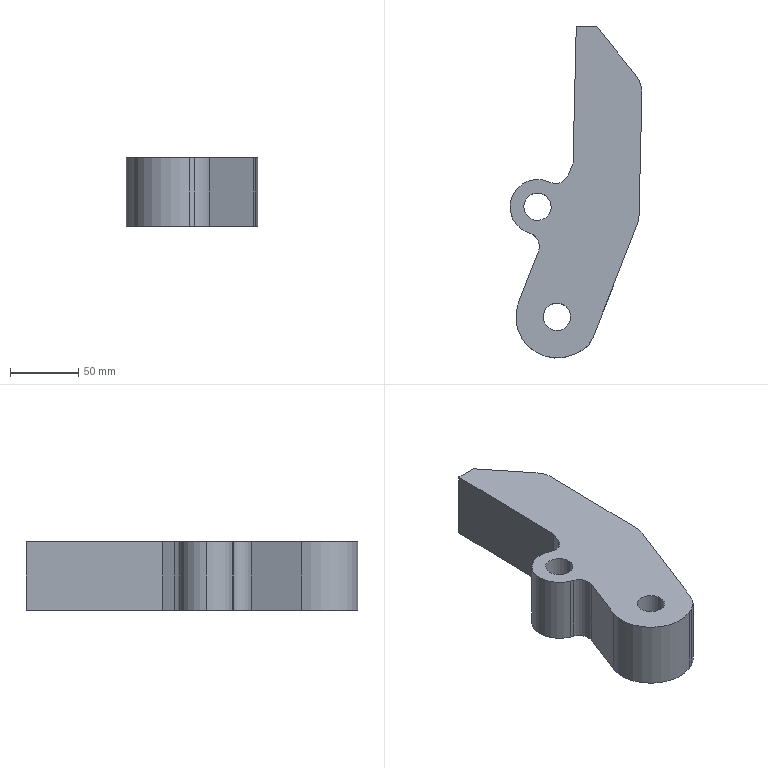Component | SolidWorks | BoxDoorCard-1 | 1 solid | 24 faces | box 96.24 x 242.36 x 50 mm | volume 653401 mm3 | cylinder 12 | plane 12 | commonest cylinder face diameters 20 x6 40 x5 60 x1
build123d program:
from build123d import *

# Parameters (mm, degrees)
BOSS_EXTRUDE1_DEPTH = 50
BOSS_EXTRUDE2_DEPTH = 50
FILLET1_R           = 10
FILLET2_R           = 20
SKETCH3_R           = 10
CUT_EXTRUDE1_DEPTH  = 255.94
SKETCH4_R           = 10
CUT_EXTRUDE2_DEPTH  = 50


with BuildPart() as part:
    # Sketch1 → Boss-Extrude1 (new body)
    with BuildSketch(Plane.XY):
        with BuildLine():
            Line((0, 0), (15, 0))
            Line((15, 0), (15, -100))
            Line((15, -100), (52.262, -202.376))
            ThreePointArc((52.262, -202.376), (44.339, -234.755), (11.393, -239.826))
            Line((11.393, -239.826), (0.1304, -234.574))
            Line((0.1304, -234.574), (-34.072, -140.605))
            Line((-34.072, -140.605), (-34.072, -40.605))
            Line((-34.072, -40.605), (0, 0))
        make_face()
    extrude(amount=BOSS_EXTRUDE1_DEPTH)

    # Sketch2 → Boss-Extrude2 (add)
    with BuildSketch(Plane.XY.offset(50)):
        with BuildLine():
            Line((21.594, -118.118), (33.341, -113.843))
            ThreePointArc((33.341, -113.843), (58.975, -125.796), (47.021, -151.431))
            Line((47.021, -151.431), (35.275, -155.706))
            Line((35.275, -155.706), (21.594, -118.118))
        make_face()
    extrude(amount=-BOSS_EXTRUDE2_DEPTH)

    # Fillet1
    fillet1_edges = [part.edges().sort_by_distance(p)[0] for p in [
        (35.275, -155.706, 25),
        (21.594, -118.118, 25),
    ]]
    fillet(fillet1_edges, radius=FILLET1_R)

    # Fillet2
    fillet2_edges = [part.edges().sort_by_distance(p)[0] for p in [
        (0.1304, -234.574, 25),
        (-34.072, -140.605, 25),
        (-34.072, -40.605, 25),
    ]]
    fillet(fillet2_edges, radius=FILLET2_R)

    # Sketch3 → Cut-Extrude1 (cut, through all)
    with BuildSketch(Plane.XY.offset(50)):
        with Locations((40.181, -132.637)):
            Circle(SKETCH3_R)
    extrude(amount=-CUT_EXTRUDE1_DEPTH, mode=Mode.SUBTRACT)

    # Sketch4 → Cut-Extrude2 (cut)
    with BuildSketch(Plane.XY.offset(50)):
        with Locations((24.071, -212.637)):
            Circle(SKETCH4_R)
    extrude(amount=-CUT_EXTRUDE2_DEPTH, mode=Mode.SUBTRACT)


solid = part.part

# Placed as in the assembly
solid = solid.moved(Location((1159.9, 1474.284, 520.114), (180, 0, -178.644)))
STEP:
#1=COLOUR_RGB('',0.7922,0.8196,0.9333);
#2=FILL_AREA_STYLE_COLOUR('',#1);
#3=FILL_AREA_STYLE('',(#2));
#4=SURFACE_STYLE_FILL_AREA(#3);
#5=SURFACE_SIDE_STYLE('',(#4));
#6=SURFACE_STYLE_USAGE(.BOTH.,#5);
#7=PRESENTATION_STYLE_ASSIGNMENT((#6));
#8=CARTESIAN_POINT('',(44.913,49.687,20.477));
#9=VERTEX_POINT('',#8);
#10=CARTESIAN_POINT('',(44.126,49.705,20.477));
#11=VERTEX_POINT('',#10);
#12=CARTESIAN_POINT('',(44.52,49.696,20.477));
#13=DIRECTION('',(-0.,-0.,-1.));
#14=DIRECTION('',(-0.9997,0.02366,0.));
#15=AXIS2_PLACEMENT_3D('',#12,#13,#14);
#16=CIRCLE('',#15,0.3937);
#17=EDGE_CURVE('',#9,#11,#16,.T.);
#18=ORIENTED_EDGE('',*,*,#17,.F.);
#19=CARTESIAN_POINT('',(44.913,49.687,18.508));
#20=VERTEX_POINT('',#19);
#21=CARTESIAN_POINT('',(44.913,49.687,20.477));
#22=DIRECTION('',(-0.,-0.,-1.));
#23=VECTOR('',#22,39.37);
#24=LINE('',#21,#23);
#25=EDGE_CURVE('',#9,#20,#24,.T.);
#26=ORIENTED_EDGE('',*,*,#25,.T.);
#27=CARTESIAN_POINT('',(44.126,49.705,18.508));
#28=VERTEX_POINT('',#27);
#29=CARTESIAN_POINT('',(44.52,49.696,18.508));
#30=DIRECTION('',(-0.,-0.,-1.));
#31=DIRECTION('',(-0.9997,0.02366,0.));
#32=AXIS2_PLACEMENT_3D('',#29,#30,#31);
#33=CIRCLE('',#32,0.3937);
#34=EDGE_CURVE('',#20,#28,#33,.T.);
#35=ORIENTED_EDGE('',*,*,#34,.T.);
#36=CARTESIAN_POINT('',(44.126,49.705,20.477));
#37=DIRECTION('',(-0.,-0.,-1.));
#38=VECTOR('',#37,39.37);
#39=LINE('',#36,#38);
#40=EDGE_CURVE('',#11,#28,#39,.T.);
#41=ORIENTED_EDGE('',*,*,#40,.F.);
#42=EDGE_LOOP('',(#18,#26,#35,#41));
#43=FACE_OUTER_BOUND('',#42,.T.);
#44=CARTESIAN_POINT('',(44.52,49.696,20.477));
#45=DIRECTION('',(-0.,-0.,-1.));
#46=DIRECTION('',(-0.9997,0.02366,0.));
#47=AXIS2_PLACEMENT_3D('',#44,#45,#46);
#48=CYLINDRICAL_SURFACE('',#47,0.3937);
#49=ADVANCED_FACE('',(#43),#48,.F.);
#50=CARTESIAN_POINT('',(44.354,52.85,20.477));
#51=VERTEX_POINT('',#50);
#52=CARTESIAN_POINT('',(43.567,52.869,20.477));
#53=VERTEX_POINT('',#52);
#54=CARTESIAN_POINT('',(43.96,52.86,20.477));
#55=DIRECTION('',(-0.,-0.,-1.));
#56=DIRECTION('',(-0.9997,0.02366,0.));
#57=AXIS2_PLACEMENT_3D('',#54,#55,#56);
#58=CIRCLE('',#57,0.3937);
#59=EDGE_CURVE('',#51,#53,#58,.T.);
#60=ORIENTED_EDGE('',*,*,#59,.F.);
#61=CARTESIAN_POINT('',(44.354,52.85,18.508));
#62=VERTEX_POINT('',#61);
#63=CARTESIAN_POINT('',(44.354,52.85,20.477));
#64=DIRECTION('',(-0.,-0.,-1.));
#65=VECTOR('',#64,39.37);
#66=LINE('',#63,#65);
#67=EDGE_CURVE('',#51,#62,#66,.T.);
#68=ORIENTED_EDGE('',*,*,#67,.T.);
#69=CARTESIAN_POINT('',(43.567,52.869,18.508));
#70=VERTEX_POINT('',#69);
#71=CARTESIAN_POINT('',(43.96,52.86,18.508));
#72=DIRECTION('',(-0.,-0.,-1.));
#73=DIRECTION('',(-0.9997,0.02366,0.));
#74=AXIS2_PLACEMENT_3D('',#71,#72,#73);
#75=CIRCLE('',#74,0.3937);
#76=EDGE_CURVE('',#62,#70,#75,.T.);
#77=ORIENTED_EDGE('',*,*,#76,.T.);
#78=CARTESIAN_POINT('',(43.567,52.869,20.477));
#79=DIRECTION('',(-0.,-0.,-1.));
#80=VECTOR('',#79,39.37);
#81=LINE('',#78,#80);
#82=EDGE_CURVE('',#53,#70,#81,.T.);
#83=ORIENTED_EDGE('',*,*,#82,.F.);
#84=EDGE_LOOP('',(#60,#68,#77,#83));
#85=FACE_OUTER_BOUND('',#84,.T.);
#86=CARTESIAN_POINT('',(43.96,52.86,20.477));
#87=DIRECTION('',(-0.,-0.,-1.));
#88=DIRECTION('',(-0.9997,0.02366,0.));
#89=AXIS2_PLACEMENT_3D('',#86,#87,#88);
#90=CYLINDRICAL_SURFACE('',#89,0.3937);
#91=ADVANCED_FACE('',(#85),#90,.F.);
#92=CARTESIAN_POINT('',(43.674,52.126,20.477));
#93=VERTEX_POINT('',#92);
#94=CARTESIAN_POINT('',(43.173,52.878,20.477));
#95=VERTEX_POINT('',#94);
#96=CARTESIAN_POINT('',(43.96,52.86,20.477));
#97=DIRECTION('',(-0.,-0.,-1.));
#98=DIRECTION('',(-0.9997,0.02366,0.));
#99=AXIS2_PLACEMENT_3D('',#96,#97,#98);
#100=CIRCLE('',#99,0.7874);
#101=EDGE_CURVE('',#93,#95,#100,.T.);
#102=ORIENTED_EDGE('',*,*,#101,.T.);
#103=CARTESIAN_POINT('',(43.173,52.878,18.508));
#104=VERTEX_POINT('',#103);
#105=CARTESIAN_POINT('',(43.173,52.878,20.477));
#106=DIRECTION('',(-0.,-0.,-1.));
#107=VECTOR('',#106,39.37);
#108=LINE('',#105,#107);
#109=EDGE_CURVE('',#95,#104,#108,.T.);
#110=ORIENTED_EDGE('',*,*,#109,.T.);
#111=CARTESIAN_POINT('',(43.674,52.126,18.508));
#112=VERTEX_POINT('',#111);
#113=CARTESIAN_POINT('',(43.96,52.86,18.508));
#114=DIRECTION('',(-0.,-0.,-1.));
#115=DIRECTION('',(-0.9997,0.02366,0.));
#116=AXIS2_PLACEMENT_3D('',#113,#114,#115);
#117=CIRCLE('',#116,0.7874);
#118=EDGE_CURVE('',#112,#104,#117,.T.);
#119=ORIENTED_EDGE('',*,*,#118,.F.);
#120=CARTESIAN_POINT('',(43.674,52.126,20.477));
#121=DIRECTION('',(-0.,-0.,-1.));
#122=VECTOR('',#121,39.37);
#123=LINE('',#120,#122);
#124=EDGE_CURVE('',#93,#112,#123,.T.);
#125=ORIENTED_EDGE('',*,*,#124,.F.);
#126=EDGE_LOOP('',(#102,#110,#119,#125));
#127=FACE_OUTER_BOUND('',#126,.T.);
#128=CARTESIAN_POINT('',(43.96,52.86,20.477));
#129=DIRECTION('',(-0.,-0.,-1.));
#130=DIRECTION('',(-0.9997,0.02366,0.));
#131=AXIS2_PLACEMENT_3D('',#128,#129,#130);
#132=CYLINDRICAL_SURFACE('',#131,0.7874);
#133=ADVANCED_FACE('',(#127),#132,.T.);
#134=CARTESIAN_POINT('',(44.849,53.78,18.508));
#135=VERTEX_POINT('',#134);
#136=CARTESIAN_POINT('',(44.982,54.121,18.508));
#137=VERTEX_POINT('',#136);
#138=CARTESIAN_POINT('',(44.982,54.121,18.508));
#139=DIRECTION('',(0.3642,0.9313,-0.));
#140=VECTOR('',#139,39.37);
#141=LINE('',#138,#140);
#142=EDGE_CURVE('',#135,#137,#141,.T.);
#143=ORIENTED_EDGE('',*,*,#142,.F.);
#144=CARTESIAN_POINT('',(44.849,53.78,20.477));
#145=VERTEX_POINT('',#144);
#146=CARTESIAN_POINT('',(44.849,53.78,18.508));
#147=DIRECTION('',(0.,0.,1.));
#148=VECTOR('',#147,39.37);
#149=LINE('',#146,#148);
#150=EDGE_CURVE('',#135,#145,#149,.T.);
#151=ORIENTED_EDGE('',*,*,#150,.T.);
#152=CARTESIAN_POINT('',(44.982,54.121,20.477));
#153=VERTEX_POINT('',#152);
#154=CARTESIAN_POINT('',(44.982,54.121,20.477));
#155=DIRECTION('',(0.3642,0.9313,-0.));
#156=VECTOR('',#155,39.37);
#157=LINE('',#154,#156);
#158=EDGE_CURVE('',#145,#153,#157,.T.);
#159=ORIENTED_EDGE('',*,*,#158,.T.);
#160=CARTESIAN_POINT('',(44.982,54.121,18.508));
#161=DIRECTION('',(0.,0.,1.));
#162=VECTOR('',#161,39.37);
#163=LINE('',#160,#162);
#164=EDGE_CURVE('',#137,#153,#163,.T.);
#165=ORIENTED_EDGE('',*,*,#164,.F.);
#166=EDGE_LOOP('',(#143,#151,#159,#165));
#167=FACE_OUTER_BOUND('',#166,.T.);
#168=CARTESIAN_POINT('',(44.982,54.121,18.508));
#169=DIRECTION('',(0.9313,-0.3642,-0.));
#170=DIRECTION('',(-0.3642,-0.9313,0.));
#171=AXIS2_PLACEMENT_3D('',#168,#169,#170);
#172=PLANE('',#171);
#173=ADVANCED_FACE('',(#167),#172,.F.);
#174=CARTESIAN_POINT('',(45.665,58.043,20.477));
#175=VERTEX_POINT('',#174);
#176=CARTESIAN_POINT('',(46.79,56.637,20.477));
#177=VERTEX_POINT('',#176);
#178=CARTESIAN_POINT('',(46.969,56.413,20.477));
#179=DIRECTION('',(0.6245,-0.781,0.));
#180=VECTOR('',#179,39.37);
#181=LINE('',#178,#180);
#182=EDGE_CURVE('',#175,#177,#181,.T.);
#183=ORIENTED_EDGE('',*,*,#182,.T.);
#184=CARTESIAN_POINT('',(46.79,56.637,18.508));
#185=VERTEX_POINT('',#184);
#186=CARTESIAN_POINT('',(46.79,56.637,18.508));
#187=DIRECTION('',(-0.,-0.,-1.));
#188=VECTOR('',#187,39.37);
#189=LINE('',#186,#188);
#190=EDGE_CURVE('',#177,#185,#189,.T.);
#191=ORIENTED_EDGE('',*,*,#190,.T.);
#192=CARTESIAN_POINT('',(45.665,58.043,18.508));
#193=VERTEX_POINT('',#192);
#194=CARTESIAN_POINT('',(46.969,56.413,18.508));
#195=DIRECTION('',(0.6245,-0.781,0.));
#196=VECTOR('',#195,39.37);
#197=LINE('',#194,#196);
#198=EDGE_CURVE('',#193,#185,#197,.T.);
#199=ORIENTED_EDGE('',*,*,#198,.F.);
#200=CARTESIAN_POINT('',(45.665,58.043,18.508));
#201=DIRECTION('',(0.,0.,1.));
#202=VECTOR('',#201,39.37);
#203=LINE('',#200,#202);
#204=EDGE_CURVE('',#193,#175,#203,.T.);
#205=ORIENTED_EDGE('',*,*,#204,.T.);
#206=EDGE_LOOP('',(#183,#191,#199,#205));
#207=FACE_OUTER_BOUND('',#206,.T.);
#208=CARTESIAN_POINT('',(46.969,56.413,18.508));
#209=DIRECTION('',(-0.781,-0.6245,0.));
#210=DIRECTION('',(-0.6245,0.781,-0.));
#211=AXIS2_PLACEMENT_3D('',#208,#209,#210);
#212=PLANE('',#211);
#213=ADVANCED_FACE('',(#207),#212,.F.);
#214=CARTESIAN_POINT('',(46.962,56.126,20.477));
#215=VERTEX_POINT('',#214);
#216=CARTESIAN_POINT('',(46.879,52.616,20.477));
#217=VERTEX_POINT('',#216);
#218=CARTESIAN_POINT('',(46.875,52.477,20.477));
#219=DIRECTION('',(-0.02366,-0.9997,0.));
#220=VECTOR('',#219,39.37);
#221=LINE('',#218,#220);
#222=EDGE_CURVE('',#215,#217,#221,.T.);
#223=ORIENTED_EDGE('',*,*,#222,.T.);
#224=CARTESIAN_POINT('',(46.879,52.616,18.508));
#225=VERTEX_POINT('',#224);
#226=CARTESIAN_POINT('',(46.879,52.616,18.508));
#227=DIRECTION('',(-0.,-0.,-1.));
#228=VECTOR('',#227,39.37);
#229=LINE('',#226,#228);
#230=EDGE_CURVE('',#217,#225,#229,.T.);
#231=ORIENTED_EDGE('',*,*,#230,.T.);
#232=CARTESIAN_POINT('',(46.962,56.126,18.508));
#233=VERTEX_POINT('',#232);
#234=CARTESIAN_POINT('',(46.875,52.477,18.508));
#235=DIRECTION('',(-0.02366,-0.9997,0.));
#236=VECTOR('',#235,39.37);
#237=LINE('',#234,#236);
#238=EDGE_CURVE('',#233,#225,#237,.T.);
#239=ORIENTED_EDGE('',*,*,#238,.F.);
#240=CARTESIAN_POINT('',(46.962,56.126,18.508));
#241=DIRECTION('',(0.,0.,1.));
#242=VECTOR('',#241,39.37);
#243=LINE('',#240,#242);
#244=EDGE_CURVE('',#233,#215,#243,.T.);
#245=ORIENTED_EDGE('',*,*,#244,.T.);
#246=EDGE_LOOP('',(#223,#231,#239,#245));
#247=FACE_OUTER_BOUND('',#246,.T.);
#248=CARTESIAN_POINT('',(46.875,52.477,18.508));
#249=DIRECTION('',(-0.9997,0.02366,0.));
#250=DIRECTION('',(0.,0.,1.));
#251=AXIS2_PLACEMENT_3D('',#248,#249,#250);
#252=PLANE('',#251);
#253=ADVANCED_FACE('',(#247),#252,.F.);
#254=CARTESIAN_POINT('',(46.825,52.348,20.477));
#255=VERTEX_POINT('',#254);
#256=CARTESIAN_POINT('',(45.56,49.114,20.477));
#257=VERTEX_POINT('',#256);
#258=CARTESIAN_POINT('',(45.442,48.81,20.477));
#259=DIRECTION('',(-0.3642,-0.9313,0.));
#260=VECTOR('',#259,39.37);
#261=LINE('',#258,#260);
#262=EDGE_CURVE('',#255,#257,#261,.T.);
#263=ORIENTED_EDGE('',*,*,#262,.T.);
#264=CARTESIAN_POINT('',(45.56,49.114,18.508));
#265=VERTEX_POINT('',#264);
#266=CARTESIAN_POINT('',(45.56,49.114,18.508));
#267=DIRECTION('',(-0.,-0.,-1.));
#268=VECTOR('',#267,39.37);
#269=LINE('',#266,#268);
#270=EDGE_CURVE('',#257,#265,#269,.T.);
#271=ORIENTED_EDGE('',*,*,#270,.T.);
#272=CARTESIAN_POINT('',(46.825,52.348,18.508));
#273=VERTEX_POINT('',#272);
#274=CARTESIAN_POINT('',(45.442,48.81,18.508));
#275=DIRECTION('',(-0.3642,-0.9313,0.));
#276=VECTOR('',#275,39.37);
#277=LINE('',#274,#276);
#278=EDGE_CURVE('',#273,#265,#277,.T.);
#279=ORIENTED_EDGE('',*,*,#278,.F.);
#280=CARTESIAN_POINT('',(46.825,52.348,18.508));
#281=DIRECTION('',(0.,0.,1.));
#282=VECTOR('',#281,39.37);
#283=LINE('',#280,#282);
#284=EDGE_CURVE('',#273,#255,#283,.T.);
#285=ORIENTED_EDGE('',*,*,#284,.T.);
#286=EDGE_LOOP('',(#263,#271,#279,#285));
#287=FACE_OUTER_BOUND('',#286,.T.);
#288=CARTESIAN_POINT('',(45.442,48.81,18.508));
#289=DIRECTION('',(-0.9313,0.3642,0.));
#290=DIRECTION('',(0.3642,0.9313,-0.));
#291=AXIS2_PLACEMENT_3D('',#288,#289,#290);
#292=PLANE('',#291);
#293=ADVANCED_FACE('',(#287),#292,.F.);
#294=CARTESIAN_POINT('',(45.143,48.679,18.508));
#295=VERTEX_POINT('',#294);
#296=CARTESIAN_POINT('',(44.994,48.614,18.508));
#297=VERTEX_POINT('',#296);
#298=CARTESIAN_POINT('',(44.994,48.614,18.508));
#299=DIRECTION('',(-0.9161,-0.4011,0.));
#300=VECTOR('',#299,39.37);
#301=LINE('',#298,#300);
#302=EDGE_CURVE('',#295,#297,#301,.T.);
#303=ORIENTED_EDGE('',*,*,#302,.F.);
#304=CARTESIAN_POINT('',(45.143,48.679,20.477));
#305=VERTEX_POINT('',#304);
#306=CARTESIAN_POINT('',(45.143,48.679,18.508));
#307=DIRECTION('',(0.,0.,1.));
#308=VECTOR('',#307,39.37);
#309=LINE('',#306,#308);
#310=EDGE_CURVE('',#295,#305,#309,.T.);
#311=ORIENTED_EDGE('',*,*,#310,.T.);
#312=CARTESIAN_POINT('',(44.994,48.614,20.477));
#313=VERTEX_POINT('',#312);
#314=CARTESIAN_POINT('',(44.994,48.614,20.477));
#315=DIRECTION('',(-0.9161,-0.4011,0.));
#316=VECTOR('',#315,39.37);
#317=LINE('',#314,#316);
#318=EDGE_CURVE('',#305,#313,#317,.T.);
#319=ORIENTED_EDGE('',*,*,#318,.T.);
#320=CARTESIAN_POINT('',(44.994,48.614,18.508));
#321=DIRECTION('',(0.,0.,1.));
#322=VECTOR('',#321,39.37);
#323=LINE('',#320,#322);
#324=EDGE_CURVE('',#297,#313,#323,.T.);
#325=ORIENTED_EDGE('',*,*,#324,.F.);
#326=EDGE_LOOP('',(#303,#311,#319,#325));
#327=FACE_OUTER_BOUND('',#326,.T.);
#328=CARTESIAN_POINT('',(44.994,48.614,18.508));
#329=DIRECTION('',(-0.4011,0.9161,-0.));
#330=DIRECTION('',(0.9161,0.4011,-0.));
#331=AXIS2_PLACEMENT_3D('',#328,#329,#330);
#332=PLANE('',#331);
#333=ADVANCED_FACE('',(#327),#332,.F.);
#334=CARTESIAN_POINT('',(43.42,50.126,20.477));
#335=VERTEX_POINT('',#334);
#336=CARTESIAN_POINT('',(44.52,49.696,20.477));
#337=DIRECTION('',(-0.,-0.,-1.));
#338=DIRECTION('',(0.9997,-0.02366,0.));
#339=AXIS2_PLACEMENT_3D('',#336,#337,#338);
#340=CIRCLE('',#339,1.181);
#341=EDGE_CURVE('',#313,#335,#340,.T.);
#342=ORIENTED_EDGE('',*,*,#341,.T.);
#343=CARTESIAN_POINT('',(43.42,50.126,18.508));
#344=VERTEX_POINT('',#343);
#345=CARTESIAN_POINT('',(43.42,50.126,18.508));
#346=DIRECTION('',(0.,0.,1.));
#347=VECTOR('',#346,39.37);
#348=LINE('',#345,#347);
#349=EDGE_CURVE('',#344,#335,#348,.T.);
#350=ORIENTED_EDGE('',*,*,#349,.F.);
#351=CARTESIAN_POINT('',(44.52,49.696,18.508));
#352=DIRECTION('',(-0.,-0.,-1.));
#353=DIRECTION('',(0.9997,-0.02366,0.));
#354=AXIS2_PLACEMENT_3D('',#351,#352,#353);
#355=CIRCLE('',#354,1.181);
#356=EDGE_CURVE('',#297,#344,#355,.T.);
#357=ORIENTED_EDGE('',*,*,#356,.F.);
#358=ORIENTED_EDGE('',*,*,#324,.T.);
#359=EDGE_LOOP('',(#342,#350,#357,#358));
#360=FACE_OUTER_BOUND('',#359,.T.);
#361=CARTESIAN_POINT('',(44.52,49.696,18.508));
#362=DIRECTION('',(0.,0.,1.));
#363=DIRECTION('',(0.9997,-0.02366,0.));
#364=AXIS2_PLACEMENT_3D('',#361,#362,#363);
#365=CYLINDRICAL_SURFACE('',#364,1.181);
#366=ADVANCED_FACE('',(#360),#365,.T.);
#367=CARTESIAN_POINT('',(43.989,51.58,20.477));
#368=VERTEX_POINT('',#367);
#369=CARTESIAN_POINT('',(44.982,54.121,20.477));
#370=DIRECTION('',(0.3642,0.9313,-0.));
#371=VECTOR('',#370,39.37);
#372=LINE('',#369,#371);
#373=EDGE_CURVE('',#335,#368,#372,.T.);
#374=ORIENTED_EDGE('',*,*,#373,.T.);
#375=CARTESIAN_POINT('',(43.989,51.58,18.508));
#376=VERTEX_POINT('',#375);
#377=CARTESIAN_POINT('',(43.989,51.58,18.508));
#378=DIRECTION('',(-0.,-0.,-1.));
#379=VECTOR('',#378,39.37);
#380=LINE('',#377,#379);
#381=EDGE_CURVE('',#368,#376,#380,.T.);
#382=ORIENTED_EDGE('',*,*,#381,.T.);
#383=CARTESIAN_POINT('',(44.982,54.121,18.508));
#384=DIRECTION('',(0.3642,0.9313,-0.));
#385=VECTOR('',#384,39.37);
#386=LINE('',#383,#385);
#387=EDGE_CURVE('',#344,#376,#386,.T.);
#388=ORIENTED_EDGE('',*,*,#387,.F.);
#389=ORIENTED_EDGE('',*,*,#349,.T.);
#390=EDGE_LOOP('',(#374,#382,#388,#389));
#391=FACE_OUTER_BOUND('',#390,.T.);
#392=CARTESIAN_POINT('',(44.982,54.121,18.508));
#393=DIRECTION('',(0.9313,-0.3642,-0.));
#394=DIRECTION('',(-0.3642,-0.9313,0.));
#395=AXIS2_PLACEMENT_3D('',#392,#393,#394);
#396=PLANE('',#395);
#397=ADVANCED_FACE('',(#391),#396,.F.);
#398=CARTESIAN_POINT('',(45.075,58.057,20.477));
#399=VERTEX_POINT('',#398);
#400=CARTESIAN_POINT('',(45.075,58.057,20.477));
#401=DIRECTION('',(0.02366,0.9997,-0.));
#402=VECTOR('',#401,39.37);
#403=LINE('',#400,#402);
#404=EDGE_CURVE('',#153,#399,#403,.T.);
#405=ORIENTED_EDGE('',*,*,#404,.T.);
#406=CARTESIAN_POINT('',(45.075,58.057,18.508));
#407=VERTEX_POINT('',#406);
#408=CARTESIAN_POINT('',(45.075,58.057,18.508));
#409=DIRECTION('',(0.,0.,1.));
#410=VECTOR('',#409,39.37);
#411=LINE('',#408,#410);
#412=EDGE_CURVE('',#407,#399,#411,.T.);
#413=ORIENTED_EDGE('',*,*,#412,.F.);
#414=CARTESIAN_POINT('',(45.075,58.057,18.508));
#415=DIRECTION('',(0.02366,0.9997,-0.));
#416=VECTOR('',#415,39.37);
#417=LINE('',#414,#416);
#418=EDGE_CURVE('',#137,#407,#417,.T.);
#419=ORIENTED_EDGE('',*,*,#418,.F.);
#420=ORIENTED_EDGE('',*,*,#164,.T.);
#421=EDGE_LOOP('',(#405,#413,#419,#420));
#422=FACE_OUTER_BOUND('',#421,.T.);
#423=CARTESIAN_POINT('',(45.075,58.057,18.508));
#424=DIRECTION('',(0.9997,-0.02366,-0.));
#425=DIRECTION('',(-0.02366,-0.9997,0.));
#426=AXIS2_PLACEMENT_3D('',#423,#424,#425);
#427=PLANE('',#426);
#428=ADVANCED_FACE('',(#422),#427,.F.);
#429=CARTESIAN_POINT('',(45.665,58.043,20.477));
#430=DIRECTION('',(0.9997,-0.02366,-0.));
#431=VECTOR('',#430,39.37);
#432=LINE('',#429,#431);
#433=EDGE_CURVE('',#399,#175,#432,.T.);
#434=ORIENTED_EDGE('',*,*,#433,.T.);
#435=ORIENTED_EDGE('',*,*,#204,.F.);
#436=CARTESIAN_POINT('',(45.665,58.043,18.508));
#437=DIRECTION('',(0.9997,-0.02366,-0.));
#438=VECTOR('',#437,39.37);
#439=LINE('',#436,#438);
#440=EDGE_CURVE('',#407,#193,#439,.T.);
#441=ORIENTED_EDGE('',*,*,#440,.F.);
#442=ORIENTED_EDGE('',*,*,#412,.T.);
#443=EDGE_LOOP('',(#434,#435,#441,#442));
#444=FACE_OUTER_BOUND('',#443,.T.);
#445=CARTESIAN_POINT('',(45.665,58.043,18.508));
#446=DIRECTION('',(-0.02366,-0.9997,0.));
#447=DIRECTION('',(0.,0.,1.));
#448=AXIS2_PLACEMENT_3D('',#445,#446,#447);
#449=PLANE('',#448);
#450=ADVANCED_FACE('',(#444),#449,.F.);
#451=CARTESIAN_POINT('',(44.52,49.696,18.508));
#452=DIRECTION('',(-0.,-0.,-1.));
#453=DIRECTION('',(-0.9997,0.02366,0.));
#454=AXIS2_PLACEMENT_3D('',#451,#452,#453);
#455=CIRCLE('',#454,0.3937);
#456=EDGE_CURVE('',#28,#20,#455,.T.);
#457=ORIENTED_EDGE('',*,*,#456,.F.);
#458=ORIENTED_EDGE('',*,*,#34,.F.);
#459=EDGE_LOOP('',(#457,#458));
#460=FACE_BOUND('',#459,.T.);
#461=CARTESIAN_POINT('',(43.96,52.86,18.508));
#462=DIRECTION('',(-0.,-0.,-1.));
#463=DIRECTION('',(-0.9997,0.02366,0.));
#464=AXIS2_PLACEMENT_3D('',#461,#462,#463);
#465=CIRCLE('',#464,0.3937);
#466=EDGE_CURVE('',#70,#62,#465,.T.);
#467=ORIENTED_EDGE('',*,*,#466,.F.);
#468=ORIENTED_EDGE('',*,*,#76,.F.);
#469=EDGE_LOOP('',(#467,#468));
#470=FACE_BOUND('',#469,.T.);
#471=ORIENTED_EDGE('',*,*,#278,.T.);
#472=CARTESIAN_POINT('',(44.827,49.401,18.508));
#473=DIRECTION('',(-0.,-0.,-1.));
#474=DIRECTION('',(0.9997,-0.02366,0.));
#475=AXIS2_PLACEMENT_3D('',#472,#473,#474);
#476=CIRCLE('',#475,0.7874);
#477=EDGE_CURVE('',#265,#295,#476,.T.);
#478=ORIENTED_EDGE('',*,*,#477,.T.);
#479=ORIENTED_EDGE('',*,*,#302,.T.);
#480=ORIENTED_EDGE('',*,*,#356,.T.);
#481=ORIENTED_EDGE('',*,*,#387,.T.);
#482=CARTESIAN_POINT('',(43.765,52.09,18.508));
#483=VERTEX_POINT('',#482);
#484=CARTESIAN_POINT('',(43.622,51.724,18.508));
#485=DIRECTION('',(0.,0.,1.));
#486=DIRECTION('',(0.9997,-0.02366,0.));
#487=AXIS2_PLACEMENT_3D('',#484,#485,#486);
#488=CIRCLE('',#487,0.3937);
#489=EDGE_CURVE('',#376,#483,#488,.T.);
#490=ORIENTED_EDGE('',*,*,#489,.T.);
#491=CARTESIAN_POINT('',(44.132,51.947,18.508));
#492=DIRECTION('',(-0.9313,0.3642,0.));
#493=VECTOR('',#492,39.37);
#494=LINE('',#491,#493);
#495=EDGE_CURVE('',#483,#112,#494,.T.);
#496=ORIENTED_EDGE('',*,*,#495,.T.);
#497=ORIENTED_EDGE('',*,*,#118,.T.);
#498=CARTESIAN_POINT('',(44.247,53.593,18.508));
#499=VERTEX_POINT('',#498);
#500=CARTESIAN_POINT('',(43.96,52.86,18.508));
#501=DIRECTION('',(-0.,-0.,-1.));
#502=DIRECTION('',(-0.9997,0.02366,0.));
#503=AXIS2_PLACEMENT_3D('',#500,#501,#502);
#504=CIRCLE('',#503,0.7874);
#505=EDGE_CURVE('',#104,#499,#504,.T.);
#506=ORIENTED_EDGE('',*,*,#505,.T.);
#507=CARTESIAN_POINT('',(44.339,53.557,18.508));
#508=VERTEX_POINT('',#507);
#509=CARTESIAN_POINT('',(44.705,53.414,18.508));
#510=DIRECTION('',(0.9313,-0.3642,-0.));
#511=VECTOR('',#510,39.37);
#512=LINE('',#509,#511);
#513=EDGE_CURVE('',#499,#508,#512,.T.);
#514=ORIENTED_EDGE('',*,*,#513,.T.);
#515=CARTESIAN_POINT('',(44.482,53.924,18.508));
#516=DIRECTION('',(0.,0.,1.));
#517=DIRECTION('',(0.9997,-0.02366,0.));
#518=AXIS2_PLACEMENT_3D('',#515,#516,#517);
#519=CIRCLE('',#518,0.3937);
#520=EDGE_CURVE('',#508,#135,#519,.T.);
#521=ORIENTED_EDGE('',*,*,#520,.T.);
#522=ORIENTED_EDGE('',*,*,#142,.T.);
#523=ORIENTED_EDGE('',*,*,#418,.T.);
#524=ORIENTED_EDGE('',*,*,#440,.T.);
#525=ORIENTED_EDGE('',*,*,#198,.T.);
#526=CARTESIAN_POINT('',(46.175,56.145,18.508));
#527=DIRECTION('',(-0.,-0.,-1.));
#528=DIRECTION('',(0.9997,-0.02366,0.));
#529=AXIS2_PLACEMENT_3D('',#526,#527,#528);
#530=CIRCLE('',#529,0.7874);
#531=EDGE_CURVE('',#185,#233,#530,.T.);
#532=ORIENTED_EDGE('',*,*,#531,.T.);
#533=ORIENTED_EDGE('',*,*,#238,.T.);
#534=CARTESIAN_POINT('',(46.092,52.634,18.508));
#535=DIRECTION('',(-0.,-0.,-1.));
#536=DIRECTION('',(0.9997,-0.02366,0.));
#537=AXIS2_PLACEMENT_3D('',#534,#535,#536);
#538=CIRCLE('',#537,0.7874);
#539=EDGE_CURVE('',#225,#273,#538,.T.);
#540=ORIENTED_EDGE('',*,*,#539,.T.);
#541=EDGE_LOOP('',(#471,#478,#479,#480,#481,#490,#496,#497,#506,#514,#521,#522,#523,#524,#525,#532,#533,#540));
#542=FACE_OUTER_BOUND('',#541,.T.);
#543=CARTESIAN_POINT('',(44.52,49.696,18.508));
#544=DIRECTION('',(0.,0.,1.));
#545=DIRECTION('',(0.9997,-0.02366,-0.));
#546=AXIS2_PLACEMENT_3D('',#543,#544,#545);
#547=PLANE('',#546);
#548=ADVANCED_FACE('',(#460,#470,#542),#547,.F.);
#549=CARTESIAN_POINT('',(44.52,49.696,20.477));
#550=DIRECTION('',(-0.,-0.,-1.));
#551=DIRECTION('',(-0.9997,0.02366,0.));
#552=AXIS2_PLACEMENT_3D('',#549,#550,#551);
#553=CIRCLE('',#552,0.3937);
#554=EDGE_CURVE('',#11,#9,#553,.T.);
#555=ORIENTED_EDGE('',*,*,#554,.T.);
#556=ORIENTED_EDGE('',*,*,#17,.T.);
#557=EDGE_LOOP('',(#555,#556));
#558=FACE_BOUND('',#557,.T.);
#559=CARTESIAN_POINT('',(43.96,52.86,20.477));
#560=DIRECTION('',(-0.,-0.,-1.));
#561=DIRECTION('',(-0.9997,0.02366,0.));
#562=AXIS2_PLACEMENT_3D('',#559,#560,#561);
#563=CIRCLE('',#562,0.3937);
#564=EDGE_CURVE('',#53,#51,#563,.T.);
#565=ORIENTED_EDGE('',*,*,#564,.T.);
#566=ORIENTED_EDGE('',*,*,#59,.T.);
#567=EDGE_LOOP('',(#565,#566));
#568=FACE_BOUND('',#567,.T.);
#569=ORIENTED_EDGE('',*,*,#318,.F.);
#570=CARTESIAN_POINT('',(44.827,49.401,20.477));
#571=DIRECTION('',(0.,0.,1.));
#572=DIRECTION('',(0.9997,-0.02366,0.));
#573=AXIS2_PLACEMENT_3D('',#570,#571,#572);
#574=CIRCLE('',#573,0.7874);
#575=EDGE_CURVE('',#305,#257,#574,.T.);
#576=ORIENTED_EDGE('',*,*,#575,.T.);
#577=ORIENTED_EDGE('',*,*,#262,.F.);
#578=CARTESIAN_POINT('',(46.092,52.634,20.477));
#579=DIRECTION('',(0.,0.,1.));
#580=DIRECTION('',(0.9997,-0.02366,0.));
#581=AXIS2_PLACEMENT_3D('',#578,#579,#580);
#582=CIRCLE('',#581,0.7874);
#583=EDGE_CURVE('',#255,#217,#582,.T.);
#584=ORIENTED_EDGE('',*,*,#583,.T.);
#585=ORIENTED_EDGE('',*,*,#222,.F.);
#586=CARTESIAN_POINT('',(46.175,56.145,20.477));
#587=DIRECTION('',(0.,0.,1.));
#588=DIRECTION('',(0.9997,-0.02366,0.));
#589=AXIS2_PLACEMENT_3D('',#586,#587,#588);
#590=CIRCLE('',#589,0.7874);
#591=EDGE_CURVE('',#215,#177,#590,.T.);
#592=ORIENTED_EDGE('',*,*,#591,.T.);
#593=ORIENTED_EDGE('',*,*,#182,.F.);
#594=ORIENTED_EDGE('',*,*,#433,.F.);
#595=ORIENTED_EDGE('',*,*,#404,.F.);
#596=ORIENTED_EDGE('',*,*,#158,.F.);
#597=CARTESIAN_POINT('',(44.339,53.557,20.477));
#598=VERTEX_POINT('',#597);
#599=CARTESIAN_POINT('',(44.482,53.924,20.477));
#600=DIRECTION('',(-0.,-0.,-1.));
#601=DIRECTION('',(0.9997,-0.02366,0.));
#602=AXIS2_PLACEMENT_3D('',#599,#600,#601);
#603=CIRCLE('',#602,0.3937);
#604=EDGE_CURVE('',#145,#598,#603,.T.);
#605=ORIENTED_EDGE('',*,*,#604,.T.);
#606=CARTESIAN_POINT('',(44.247,53.593,20.477));
#607=VERTEX_POINT('',#606);
#608=CARTESIAN_POINT('',(44.705,53.414,20.477));
#609=DIRECTION('',(0.9313,-0.3642,-0.));
#610=VECTOR('',#609,39.37);
#611=LINE('',#608,#610);
#612=EDGE_CURVE('',#607,#598,#611,.T.);
#613=ORIENTED_EDGE('',*,*,#612,.F.);
#614=CARTESIAN_POINT('',(43.96,52.86,20.477));
#615=DIRECTION('',(-0.,-0.,-1.));
#616=DIRECTION('',(-0.9997,0.02366,0.));
#617=AXIS2_PLACEMENT_3D('',#614,#615,#616);
#618=CIRCLE('',#617,0.7874);
#619=EDGE_CURVE('',#95,#607,#618,.T.);
#620=ORIENTED_EDGE('',*,*,#619,.F.);
#621=ORIENTED_EDGE('',*,*,#101,.F.);
#622=CARTESIAN_POINT('',(43.765,52.09,20.477));
#623=VERTEX_POINT('',#622);
#624=CARTESIAN_POINT('',(44.132,51.947,20.477));
#625=DIRECTION('',(-0.9313,0.3642,0.));
#626=VECTOR('',#625,39.37);
#627=LINE('',#624,#626);
#628=EDGE_CURVE('',#623,#93,#627,.T.);
#629=ORIENTED_EDGE('',*,*,#628,.F.);
#630=CARTESIAN_POINT('',(43.622,51.724,20.477));
#631=DIRECTION('',(-0.,-0.,-1.));
#632=DIRECTION('',(0.9997,-0.02366,0.));
#633=AXIS2_PLACEMENT_3D('',#630,#631,#632);
#634=CIRCLE('',#633,0.3937);
#635=EDGE_CURVE('',#623,#368,#634,.T.);
#636=ORIENTED_EDGE('',*,*,#635,.T.);
#637=ORIENTED_EDGE('',*,*,#373,.F.);
#638=ORIENTED_EDGE('',*,*,#341,.F.);
#639=EDGE_LOOP('',(#569,#576,#577,#584,#585,#592,#593,#594,#595,#596,#605,#613,#620,#621,#629,#636,#637,#638));
#640=FACE_OUTER_BOUND('',#639,.T.);
#641=CARTESIAN_POINT('',(44.52,49.696,20.477));
#642=DIRECTION('',(0.,0.,1.));
#643=DIRECTION('',(0.9997,-0.02366,-0.));
#644=AXIS2_PLACEMENT_3D('',#641,#642,#643);
#645=PLANE('',#644);
#646=ADVANCED_FACE('',(#558,#568,#640),#645,.T.);
#647=ORIENTED_EDGE('',*,*,#612,.T.);
#648=CARTESIAN_POINT('',(44.339,53.557,20.477));
#649=DIRECTION('',(-0.,-0.,-1.));
#650=VECTOR('',#649,39.37);
#651=LINE('',#648,#650);
#652=EDGE_CURVE('',#598,#508,#651,.T.);
#653=ORIENTED_EDGE('',*,*,#652,.T.);
#654=ORIENTED_EDGE('',*,*,#513,.F.);
#655=CARTESIAN_POINT('',(44.247,53.593,20.477));
#656=DIRECTION('',(-0.,-0.,-1.));
#657=VECTOR('',#656,39.37);
#658=LINE('',#655,#657);
#659=EDGE_CURVE('',#607,#499,#658,.T.);
#660=ORIENTED_EDGE('',*,*,#659,.F.);
#661=EDGE_LOOP('',(#647,#653,#654,#660));
#662=FACE_OUTER_BOUND('',#661,.T.);
#663=CARTESIAN_POINT('',(44.705,53.414,20.477));
#664=DIRECTION('',(0.3642,0.9313,-0.));
#665=DIRECTION('',(0.9313,-0.3642,-0.));
#666=AXIS2_PLACEMENT_3D('',#663,#664,#665);
#667=PLANE('',#666);
#668=ADVANCED_FACE('',(#662),#667,.T.);
#669=ORIENTED_EDGE('',*,*,#109,.F.);
#670=ORIENTED_EDGE('',*,*,#619,.T.);
#671=ORIENTED_EDGE('',*,*,#659,.T.);
#672=ORIENTED_EDGE('',*,*,#505,.F.);
#673=EDGE_LOOP('',(#669,#670,#671,#672));
#674=FACE_OUTER_BOUND('',#673,.T.);
#675=CARTESIAN_POINT('',(43.96,52.86,20.477));
#676=DIRECTION('',(-0.,-0.,-1.));
#677=DIRECTION('',(-0.9997,0.02366,0.));
#678=AXIS2_PLACEMENT_3D('',#675,#676,#677);
#679=CYLINDRICAL_SURFACE('',#678,0.7874);
#680=ADVANCED_FACE('',(#674),#679,.T.);
#681=ORIENTED_EDGE('',*,*,#495,.F.);
#682=CARTESIAN_POINT('',(43.765,52.09,20.477));
#683=DIRECTION('',(0.,0.,1.));
#684=VECTOR('',#683,39.37);
#685=LINE('',#682,#684);
#686=EDGE_CURVE('',#483,#623,#685,.T.);
#687=ORIENTED_EDGE('',*,*,#686,.T.);
#688=ORIENTED_EDGE('',*,*,#628,.T.);
#689=ORIENTED_EDGE('',*,*,#124,.T.);
#690=EDGE_LOOP('',(#681,#687,#688,#689));
#691=FACE_OUTER_BOUND('',#690,.T.);
#692=CARTESIAN_POINT('',(44.132,51.947,20.477));
#693=DIRECTION('',(-0.3642,-0.9313,0.));
#694=DIRECTION('',(-0.9313,0.3642,0.));
#695=AXIS2_PLACEMENT_3D('',#692,#693,#694);
#696=PLANE('',#695);
#697=ADVANCED_FACE('',(#691),#696,.T.);
#698=ORIENTED_EDGE('',*,*,#604,.F.);
#699=ORIENTED_EDGE('',*,*,#150,.F.);
#700=ORIENTED_EDGE('',*,*,#520,.F.);
#701=ORIENTED_EDGE('',*,*,#652,.F.);
#702=EDGE_LOOP('',(#698,#699,#700,#701));
#703=FACE_OUTER_BOUND('',#702,.T.);
#704=CARTESIAN_POINT('',(44.482,53.924,20.477));
#705=DIRECTION('',(-0.,-0.,-1.));
#706=DIRECTION('',(-0.9997,0.02366,0.));
#707=AXIS2_PLACEMENT_3D('',#704,#705,#706);
#708=CYLINDRICAL_SURFACE('',#707,0.3937);
#709=ADVANCED_FACE('',(#703),#708,.F.);
#710=ORIENTED_EDGE('',*,*,#635,.F.);
#711=ORIENTED_EDGE('',*,*,#686,.F.);
#712=ORIENTED_EDGE('',*,*,#489,.F.);
#713=ORIENTED_EDGE('',*,*,#381,.F.);
#714=EDGE_LOOP('',(#710,#711,#712,#713));
#715=FACE_OUTER_BOUND('',#714,.T.);
#716=CARTESIAN_POINT('',(43.622,51.724,18.508));
#717=DIRECTION('',(-0.,-0.,-1.));
#718=DIRECTION('',(-0.9997,0.02366,0.));
#719=AXIS2_PLACEMENT_3D('',#716,#717,#718);
#720=CYLINDRICAL_SURFACE('',#719,0.3937);
#721=ADVANCED_FACE('',(#715),#720,.F.);
#722=ORIENTED_EDGE('',*,*,#477,.F.);
#723=ORIENTED_EDGE('',*,*,#270,.F.);
#724=ORIENTED_EDGE('',*,*,#575,.F.);
#725=ORIENTED_EDGE('',*,*,#310,.F.);
#726=EDGE_LOOP('',(#722,#723,#724,#725));
#727=FACE_OUTER_BOUND('',#726,.T.);
#728=CARTESIAN_POINT('',(44.827,49.401,18.508));
#729=DIRECTION('',(0.,0.,1.));
#730=DIRECTION('',(0.9997,-0.02366,0.));
#731=AXIS2_PLACEMENT_3D('',#728,#729,#730);
#732=CYLINDRICAL_SURFACE('',#731,0.7874);
#733=ADVANCED_FACE('',(#727),#732,.T.);
#734=ORIENTED_EDGE('',*,*,#539,.F.);
#735=ORIENTED_EDGE('',*,*,#230,.F.);
#736=ORIENTED_EDGE('',*,*,#583,.F.);
#737=ORIENTED_EDGE('',*,*,#284,.F.);
#738=EDGE_LOOP('',(#734,#735,#736,#737));
#739=FACE_OUTER_BOUND('',#738,.T.);
#740=CARTESIAN_POINT('',(46.092,52.634,18.508));
#741=DIRECTION('',(0.,0.,1.));
#742=DIRECTION('',(0.9997,-0.02366,0.));
#743=AXIS2_PLACEMENT_3D('',#740,#741,#742);
#744=CYLINDRICAL_SURFACE('',#743,0.7874);
#745=ADVANCED_FACE('',(#739),#744,.T.);
#746=ORIENTED_EDGE('',*,*,#531,.F.);
#747=ORIENTED_EDGE('',*,*,#190,.F.);
#748=ORIENTED_EDGE('',*,*,#591,.F.);
#749=ORIENTED_EDGE('',*,*,#244,.F.);
#750=EDGE_LOOP('',(#746,#747,#748,#749));
#751=FACE_OUTER_BOUND('',#750,.T.);
#752=CARTESIAN_POINT('',(46.175,56.145,18.508));
#753=DIRECTION('',(0.,0.,1.));
#754=DIRECTION('',(0.9997,-0.02366,0.));
#755=AXIS2_PLACEMENT_3D('',#752,#753,#754);
#756=CYLINDRICAL_SURFACE('',#755,0.7874);
#757=ADVANCED_FACE('',(#751),#756,.T.);
#758=ORIENTED_EDGE('',*,*,#67,.F.);
#759=ORIENTED_EDGE('',*,*,#564,.F.);
#760=ORIENTED_EDGE('',*,*,#82,.T.);
#761=ORIENTED_EDGE('',*,*,#466,.T.);
#762=EDGE_LOOP('',(#758,#759,#760,#761));
#763=FACE_OUTER_BOUND('',#762,.T.);
#764=CARTESIAN_POINT('',(43.96,52.86,20.477));
#765=DIRECTION('',(-0.,-0.,-1.));
#766=DIRECTION('',(-0.9997,0.02366,0.));
#767=AXIS2_PLACEMENT_3D('',#764,#765,#766);
#768=CYLINDRICAL_SURFACE('',#767,0.3937);
#769=ADVANCED_FACE('',(#763),#768,.F.);
#770=ORIENTED_EDGE('',*,*,#25,.F.);
#771=ORIENTED_EDGE('',*,*,#554,.F.);
#772=ORIENTED_EDGE('',*,*,#40,.T.);
#773=ORIENTED_EDGE('',*,*,#456,.T.);
#774=EDGE_LOOP('',(#770,#771,#772,#773));
#775=FACE_OUTER_BOUND('',#774,.T.);
#776=CARTESIAN_POINT('',(44.52,49.696,20.477));
#777=DIRECTION('',(-0.,-0.,-1.));
#778=DIRECTION('',(-0.9997,0.02366,0.));
#779=AXIS2_PLACEMENT_3D('',#776,#777,#778);
#780=CYLINDRICAL_SURFACE('',#779,0.3937);
#781=ADVANCED_FACE('',(#775),#780,.F.);
#782=CLOSED_SHELL('',(#49,#91,#133,#173,#213,#253,#293,#333,#366,#397,#428,#450,#548,#646,#668,#680,#697,#709,#721,#733,#745,#757,#769,#781));
#783=MANIFOLD_SOLID_BREP('',#782);
#784=STYLED_ITEM('',(#7),#783);
#785=(LENGTH_UNIT()NAMED_UNIT(*)SI_UNIT($,.METRE.));
#786=LENGTH_MEASURE_WITH_UNIT(LENGTH_MEASURE(0.0254),#785);
#787=DIMENSIONAL_EXPONENTS(1.,0.,0.,0.,0.,0.,0.);
#788=(CONVERSION_BASED_UNIT('',#786)LENGTH_UNIT()NAMED_UNIT(#787));
#789=UNCERTAINTY_MEASURE_WITH_UNIT(LENGTH_MEASURE(0.00001),#788,'','');
#790=(NAMED_UNIT(*)PLANE_ANGLE_UNIT()SI_UNIT($,.RADIAN.));
#791=(NAMED_UNIT(*)SI_UNIT($,.STERADIAN.)SOLID_ANGLE_UNIT());
#792=(GEOMETRIC_REPRESENTATION_CONTEXT(3)GLOBAL_UNCERTAINTY_ASSIGNED_CONTEXT((#789))GLOBAL_UNIT_ASSIGNED_CONTEXT((#788,#790,#791))REPRESENTATION_CONTEXT('',''));
#793=MECHANICAL_DESIGN_GEOMETRIC_PRESENTATION_REPRESENTATION('',(#784),#792);
#794=CARTESIAN_POINT('',(0.,0.,0.));
#795=DIRECTION('',(0.,0.,1.));
#796=DIRECTION('',(1.,0.,0.));
#797=AXIS2_PLACEMENT_3D('',#794,#795,#796);
#798=(LENGTH_UNIT()NAMED_UNIT(*)SI_UNIT($,.METRE.));
#799=LENGTH_MEASURE_WITH_UNIT(LENGTH_MEASURE(0.0254),#798);
#800=DIMENSIONAL_EXPONENTS(1.,0.,0.,0.,0.,0.,0.);
#801=(CONVERSION_BASED_UNIT('',#799)LENGTH_UNIT()NAMED_UNIT(#800));
#802=UNCERTAINTY_MEASURE_WITH_UNIT(LENGTH_MEASURE(0.00001),#801,'','');
#803=(NAMED_UNIT(*)PLANE_ANGLE_UNIT()SI_UNIT($,.RADIAN.));
#804=(NAMED_UNIT(*)SI_UNIT($,.STERADIAN.)SOLID_ANGLE_UNIT());
#805=(GEOMETRIC_REPRESENTATION_CONTEXT(3)GLOBAL_UNCERTAINTY_ASSIGNED_CONTEXT((#802))GLOBAL_UNIT_ASSIGNED_CONTEXT((#801,#803,#804))REPRESENTATION_CONTEXT('',''));
#806=ADVANCED_BREP_SHAPE_REPRESENTATION('',(#783,#797),#805);
#807=PRESENTATION_LAYER_ASSIGNMENT('','',(#784));